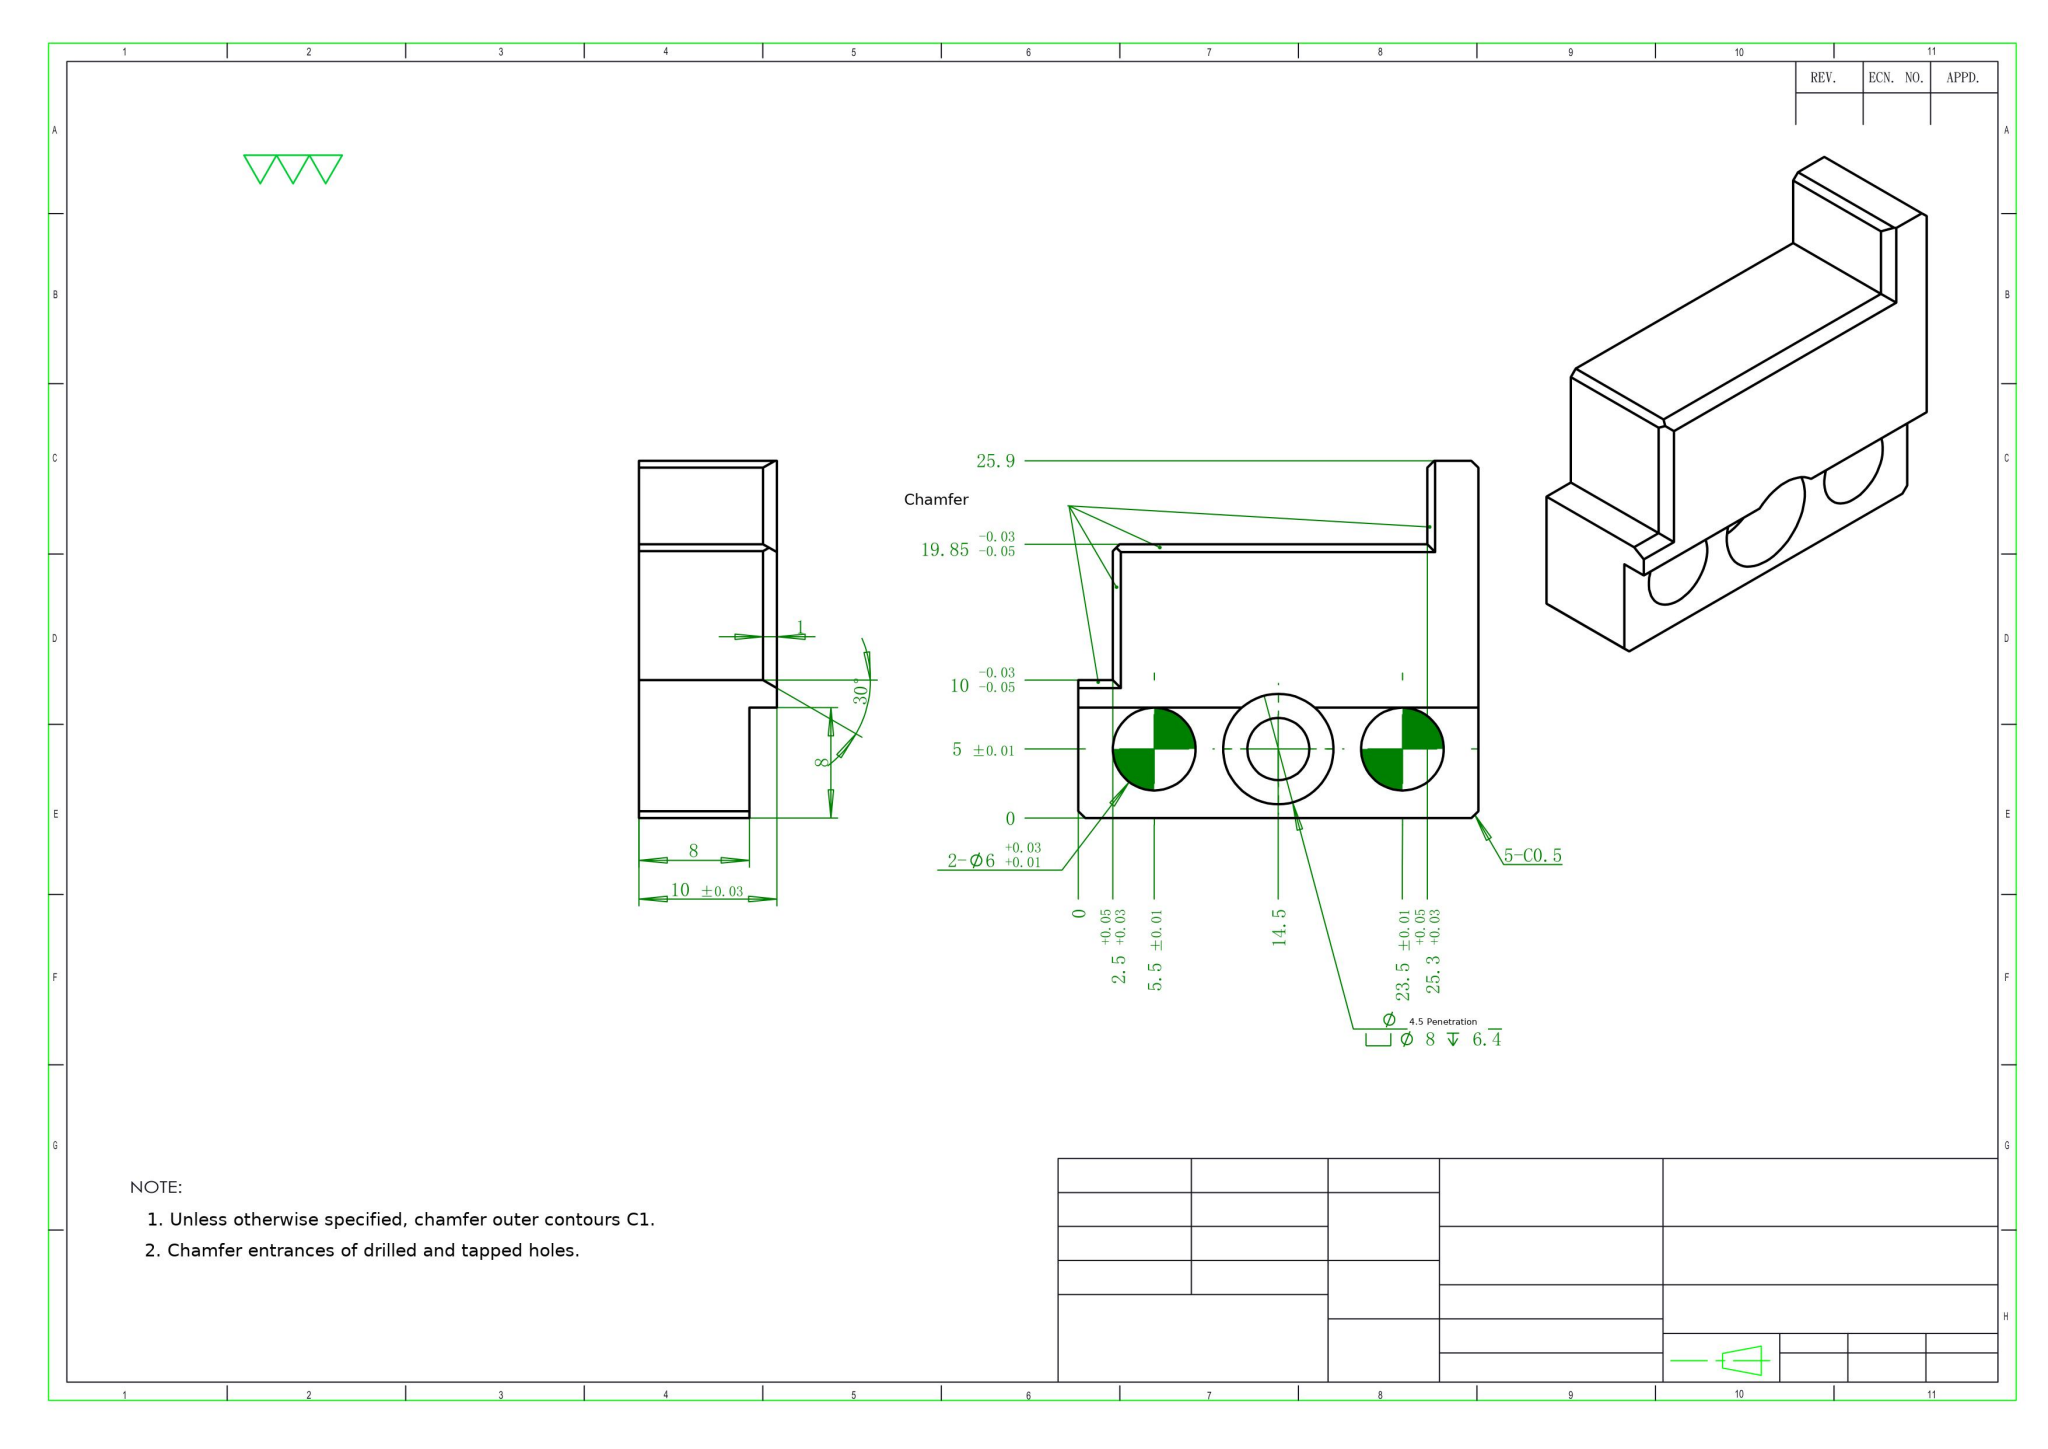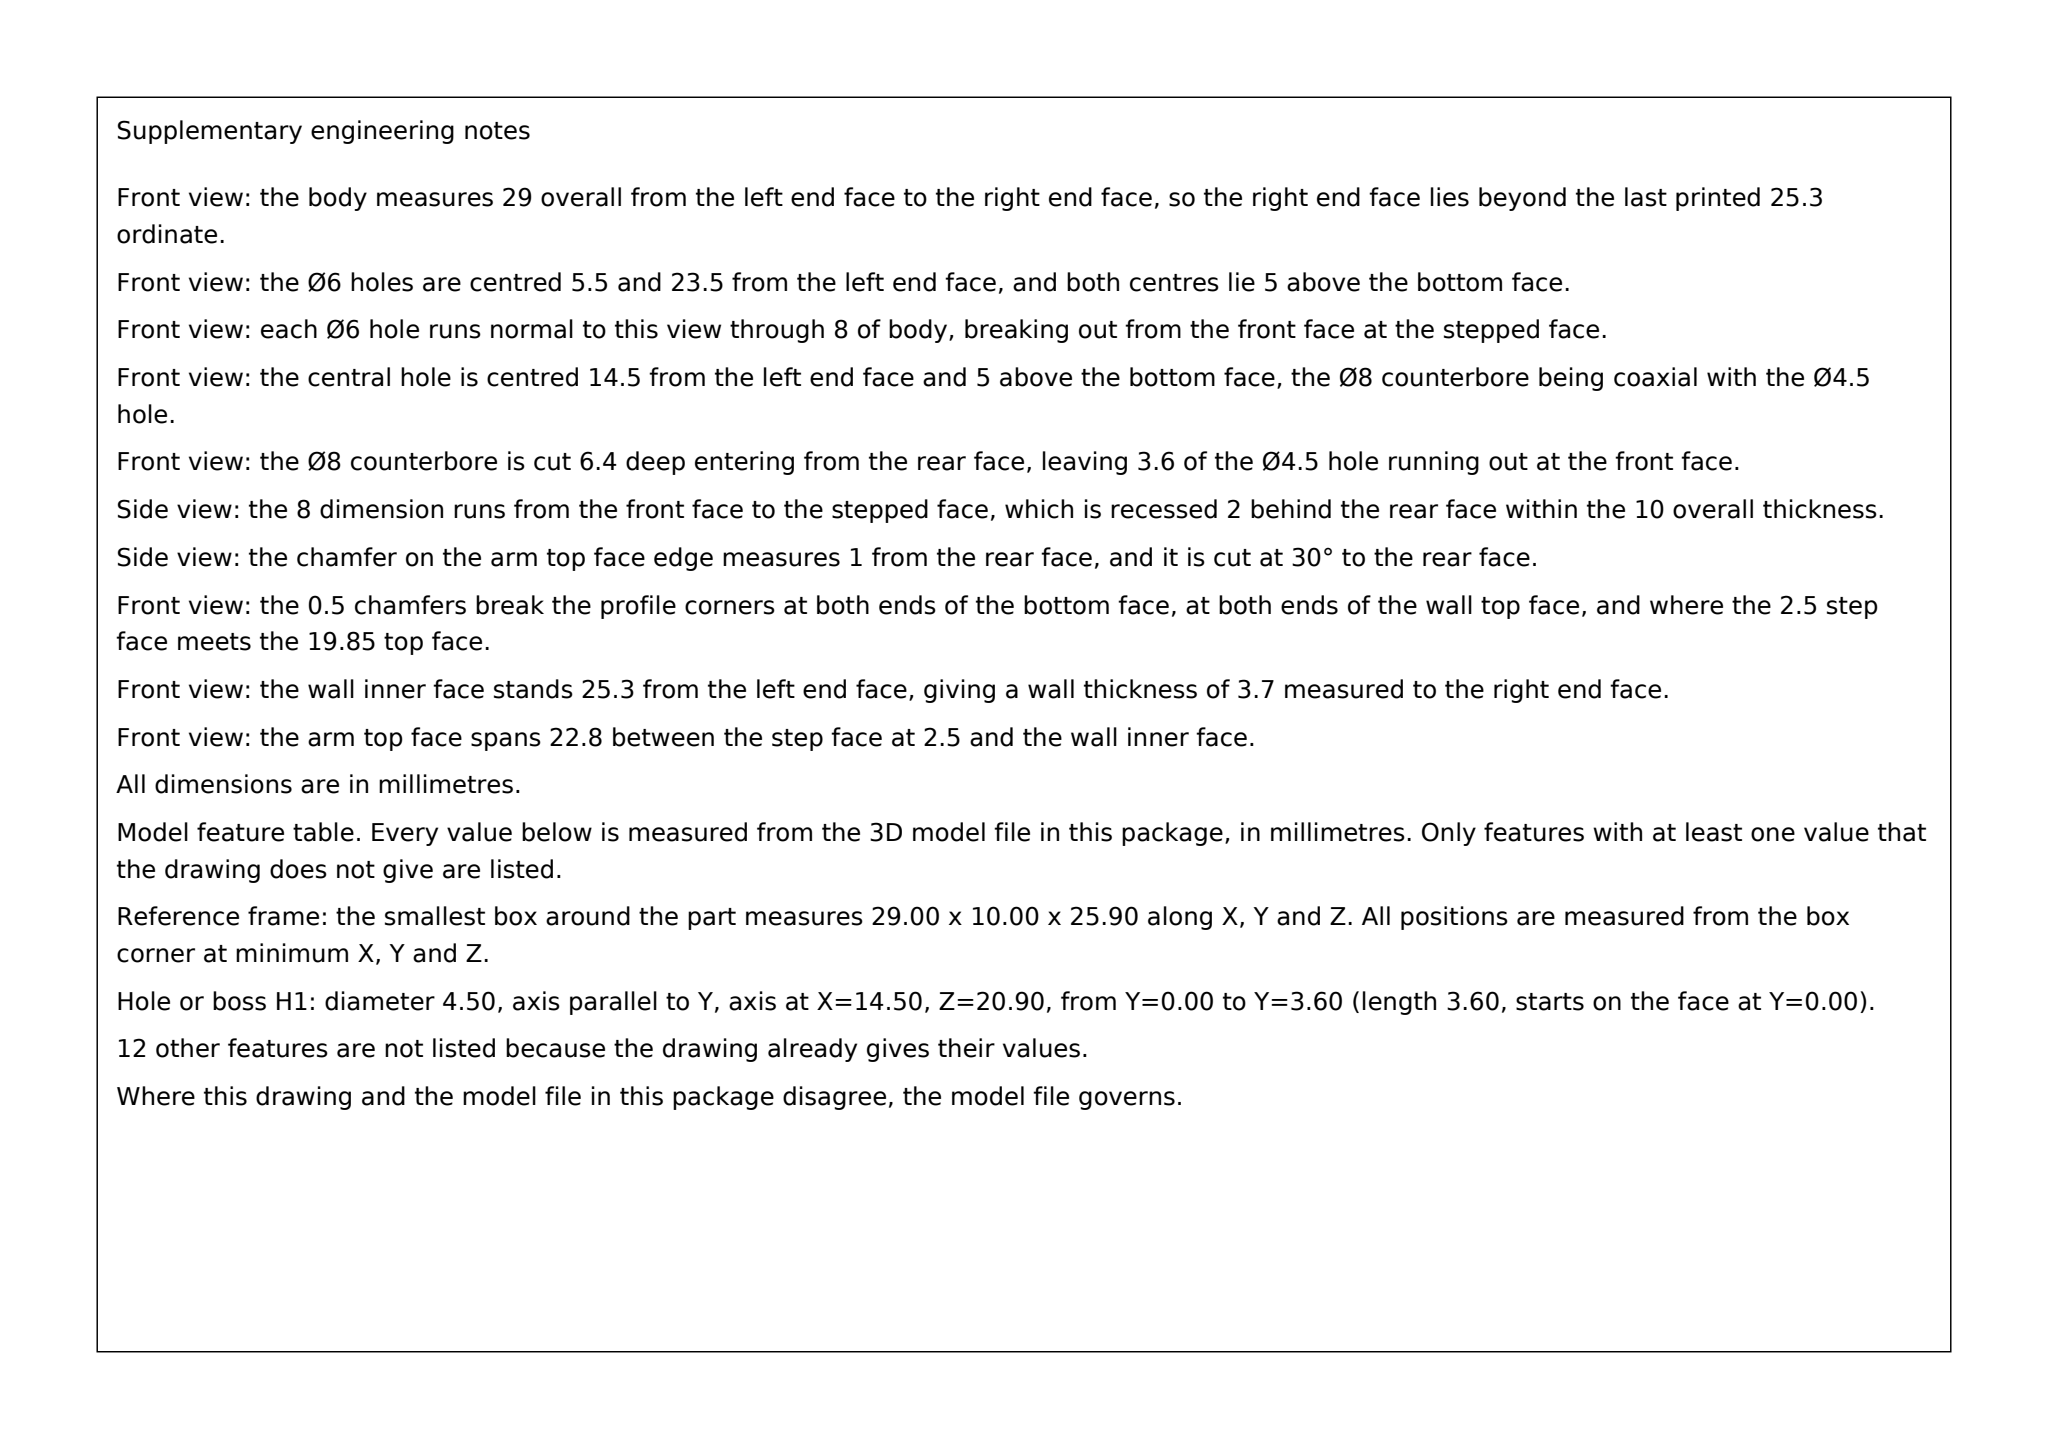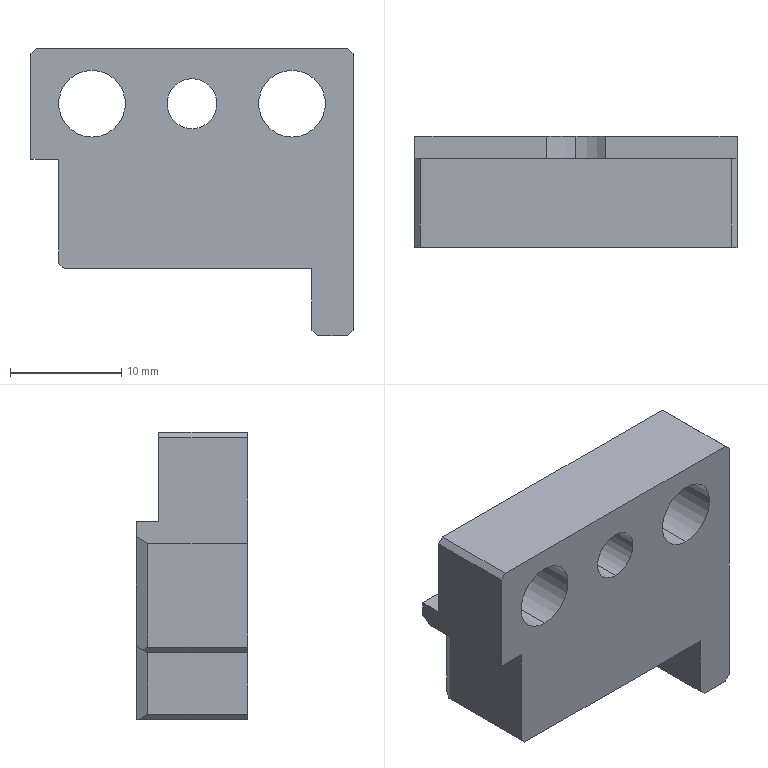Part | SolidWorks | mm | 1 solid | 31 faces | box 29 x 10 x 25.9 mm | volume 4514 mm3 | plane 23 | cylinder 8 | commonest cylinder face diameters 6 x4 8 x2 4.5 x2
Drawing notes:
FRONT VIEW: ADD ORDINATE 29 TO RH END FACE; RH RISE 3.7 WIDE | from the solid: bbox X = 29.0; x-planes at 25.3 and 29.0 -> 29.0-25.3 = 3.7 wide rise
2-Ø6 +0.03/+0.01 DP 8 FROM FRONT FACE (SAME FACE AS Ø8 C'BORE) | from the solid: cyl dia 6.0, axis y, len 8.0 at x=5.5 & x=23.5, z=20.9; y-planes 0/8.0/10.0; Ø8 c'bore len 6.4 same side
build123d program:
from build123d import *
from OCP.BRepFilletAPI import BRepFilletAPI_MakeChamfer

# Parameters (mm, degrees)
BOSS_EXTRUDE1_DEPTH                             = 10
CHAMFER1_SIZE                                   = 1
CHAMFER1_SIZE2                                  = 0.5774
M4_HEX_SOCKET_HEAD_CAP_SCREW_CBORE1_D           = 4.5
M4_HEX_SOCKET_HEAD_CAP_SCREW_CBORE1_CBORE_D     = 8
M4_HEX_SOCKET_HEAD_CAP_SCREW_CBORE1_CBORE_DEPTH = 6.4
F_6_0_6_DIAMETER_HOLE1_D                        = 6
CHAMFER2_SIZE                                   = 0.5
SKETCH7_W                                       = 29
SKETCH7_H                                       = 8
CUT_EXTRUDE1_DEPTH                              = 2


with BuildPart() as part:
    # Sketch1 → Boss-Extrude1 (new body)
    with BuildSketch(Plane(origin=(0, 0, 0), x_dir=(1, 0, 0), z_dir=(0, 1, 0))):
        Polygon((0, 0), (0, 10), (2.5, 10), (2.5, 19.85), (25.3, 19.85), (25.3, 25.9), (29, 25.9), (29, 0), align=None)
    extrude(amount=BOSS_EXTRUDE1_DEPTH)

    # Chamfer1: one chamfer whose edges measure the first distance from different faces: ONE call of the kernel's chamfer builder (chamfer() names one face for all edges)
    chamfer1_edges_1 = [part.edges().sort_by_distance(p)[0] for p in [
        (25.3, 10, -22.875),
    ]]
    chamfer1_side_1 = [part.faces().sort_by_distance(p)[0] for p in [
        (25.3, 5, -22.875),
    ]]
    chamfer1_edges_2 = [part.edges().sort_by_distance(p)[0] for p in [
        (13.9, 10, -19.85),
    ]]
    chamfer1_side_2 = [part.faces().sort_by_distance(p)[0] for p in [
        (13.9, 5, -19.85),
    ]]
    chamfer1_edges_3 = [part.edges().sort_by_distance(p)[0] for p in [
        (2.5, 10, -14.925),
    ]]
    chamfer1_side_3 = [part.faces().sort_by_distance(p)[0] for p in [
        (2.5, 5, -14.925),
    ]]
    chamfer1_edges_4 = [part.edges().sort_by_distance(p)[0] for p in [
        (1.25, 10, -10),
    ]]
    chamfer1_side_4 = [part.faces().sort_by_distance(p)[0] for p in [
        (1.25, 5, -10),
    ]]
    chamfer1 = BRepFilletAPI_MakeChamfer(part.part.solid().wrapped)
    for e in chamfer1_edges_1:
        chamfer1.Add(CHAMFER1_SIZE, CHAMFER1_SIZE2, e.wrapped, chamfer1_side_1[0].wrapped)  # the first distance lies on this face
    for e in chamfer1_edges_2:
        chamfer1.Add(CHAMFER1_SIZE, CHAMFER1_SIZE2, e.wrapped, chamfer1_side_2[0].wrapped)  # the first distance lies on this face
    for e in chamfer1_edges_3:
        chamfer1.Add(CHAMFER1_SIZE, CHAMFER1_SIZE2, e.wrapped, chamfer1_side_3[0].wrapped)  # the first distance lies on this face
    for e in chamfer1_edges_4:
        chamfer1.Add(CHAMFER1_SIZE, CHAMFER1_SIZE2, e.wrapped, chamfer1_side_4[0].wrapped)  # the first distance lies on this face
    add(Compound.cast(chamfer1.Shape()), mode=Mode.REPLACE)

    # M4 Hex Socket Head Cap Screw CBORE1 (through all)
    with Locations(Plane(origin=(0, 10, 0), x_dir=(1, 0, 0), z_dir=(0, 1, 0))):
        with Locations((14.5, 5)):
            CounterBoreHole(M4_HEX_SOCKET_HEAD_CAP_SCREW_CBORE1_D / 2, M4_HEX_SOCKET_HEAD_CAP_SCREW_CBORE1_CBORE_D / 2, M4_HEX_SOCKET_HEAD_CAP_SCREW_CBORE1_CBORE_DEPTH)

    # 6.0 _6_ Diameter Hole1 (through all)
    with Locations(Plane(origin=(0, 10, 0), x_dir=(1, 0, 0), z_dir=(0, 1, 0))):
        with Locations((5.5, 5), (23.5, 5)):
            Hole(F_6_0_6_DIAMETER_HOLE1_D / 2)

    # Chamfer2
    chamfer2_edges = [part.edges().sort_by_distance(p)[0] for p in [
        (0, 5, 0),
        (29, 5, -25.9),
        (29, 5, 0),
        (25.3, 4.5, -25.9),
        (2.5, 4.5, -19.85),
    ]]
    chamfer(chamfer2_edges, length=CHAMFER2_SIZE)

    # Sketch7 → Cut-Extrude1 (cut)
    with BuildSketch(Plane(origin=(0, 10, 0), x_dir=(1, 0, 0), z_dir=(0, 1, 0))):
        with Locations((14.5, 4)):
            Rectangle(SKETCH7_W, SKETCH7_H)
    extrude(amount=-CUT_EXTRUDE1_DEPTH, mode=Mode.SUBTRACT)


solid = part.part